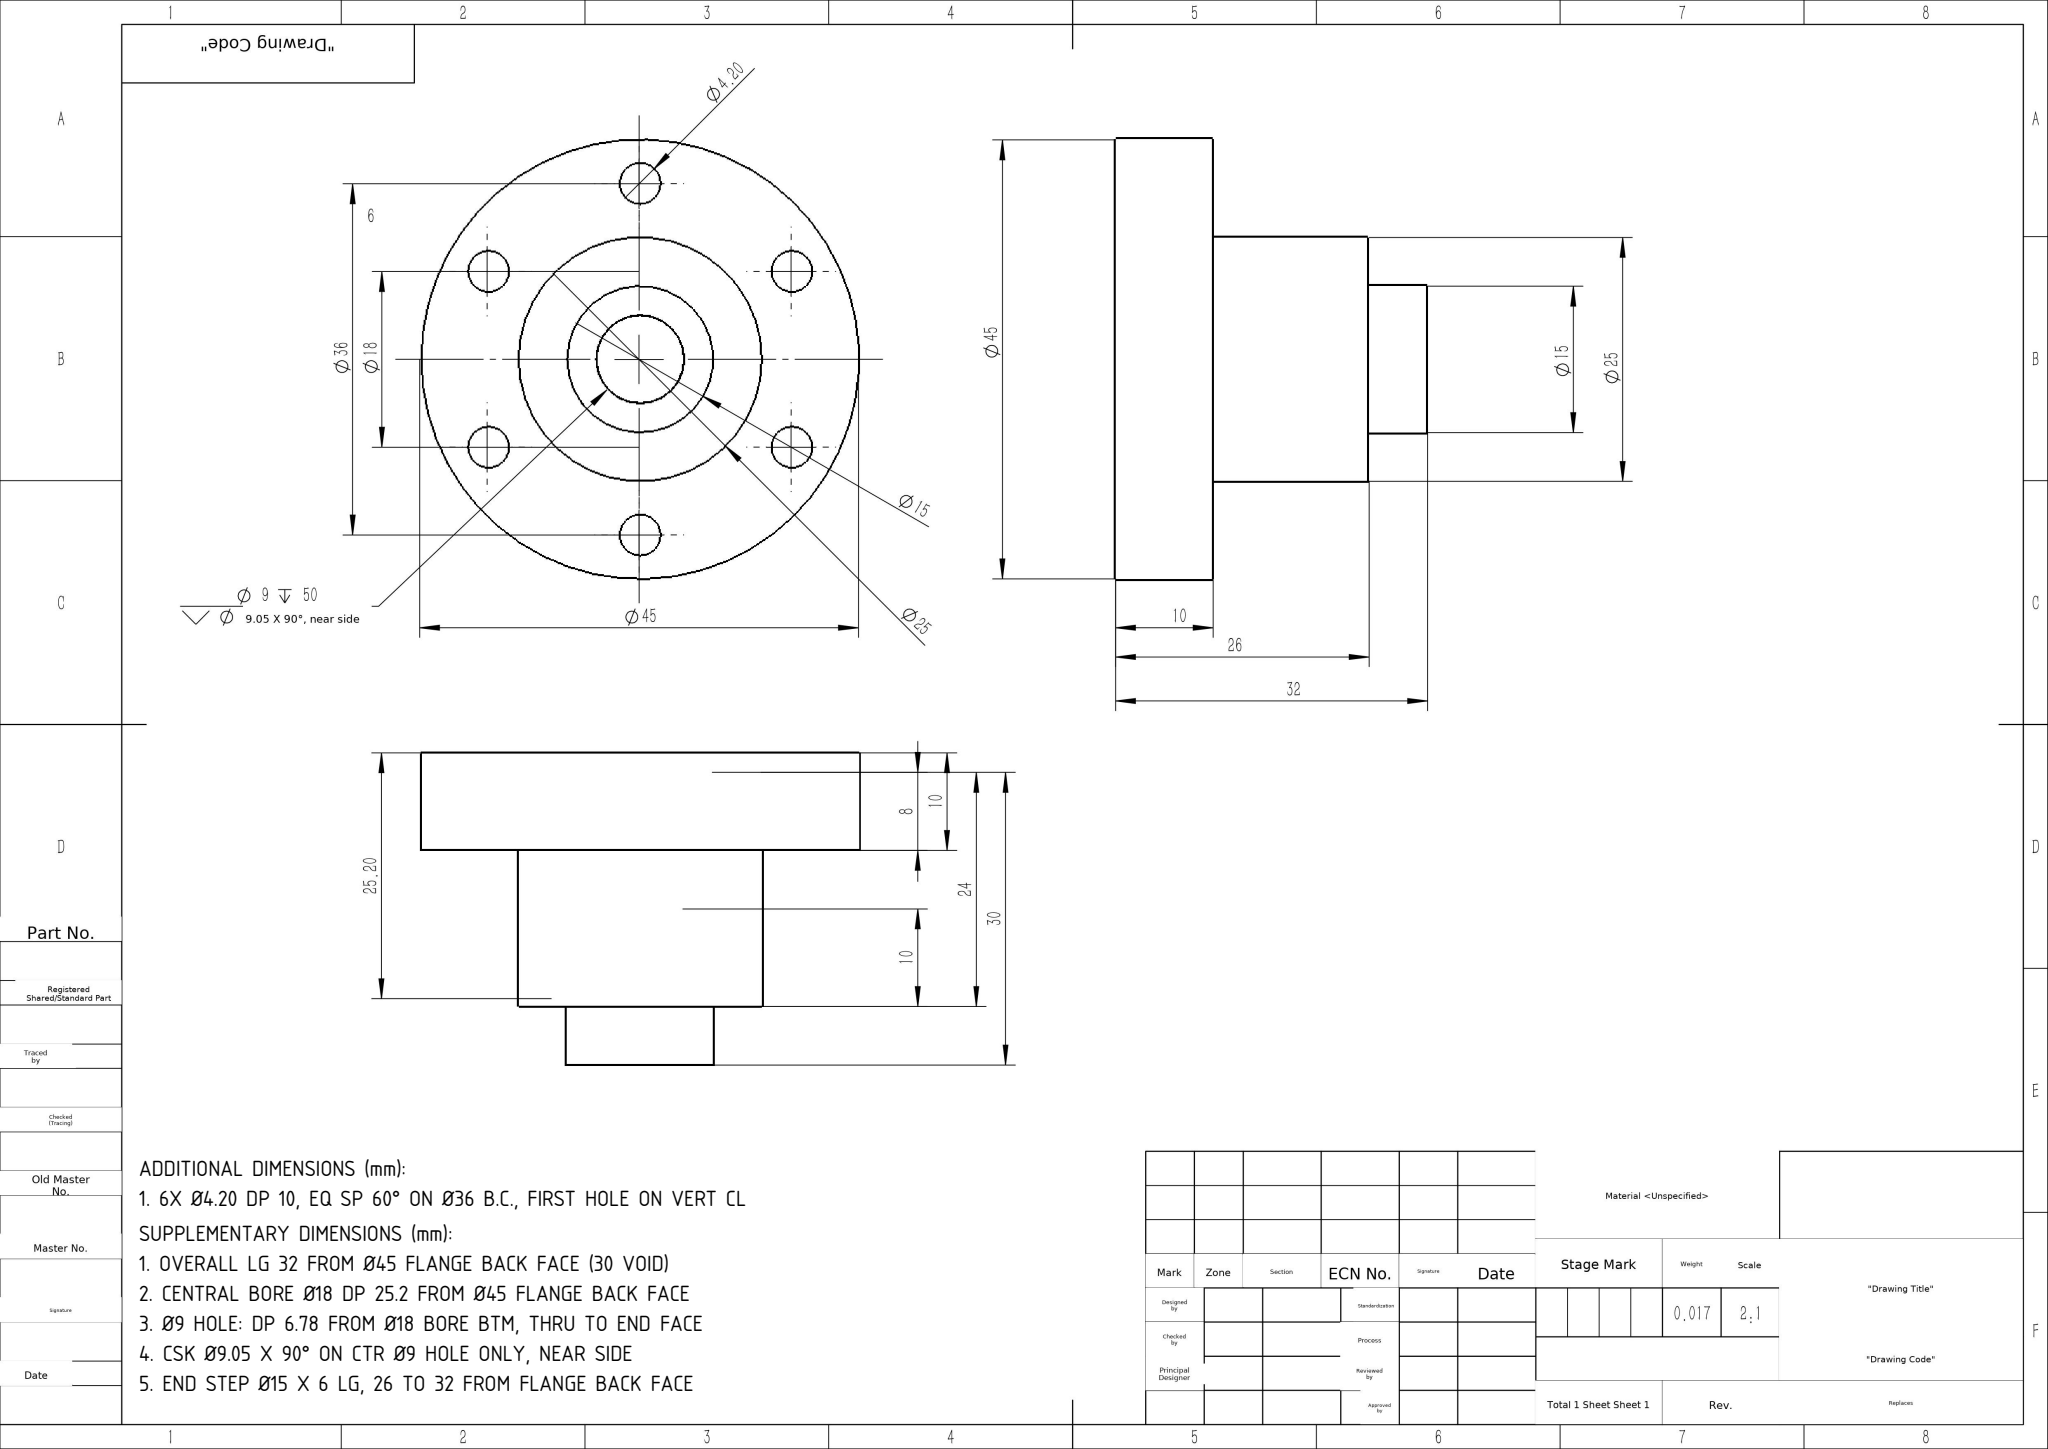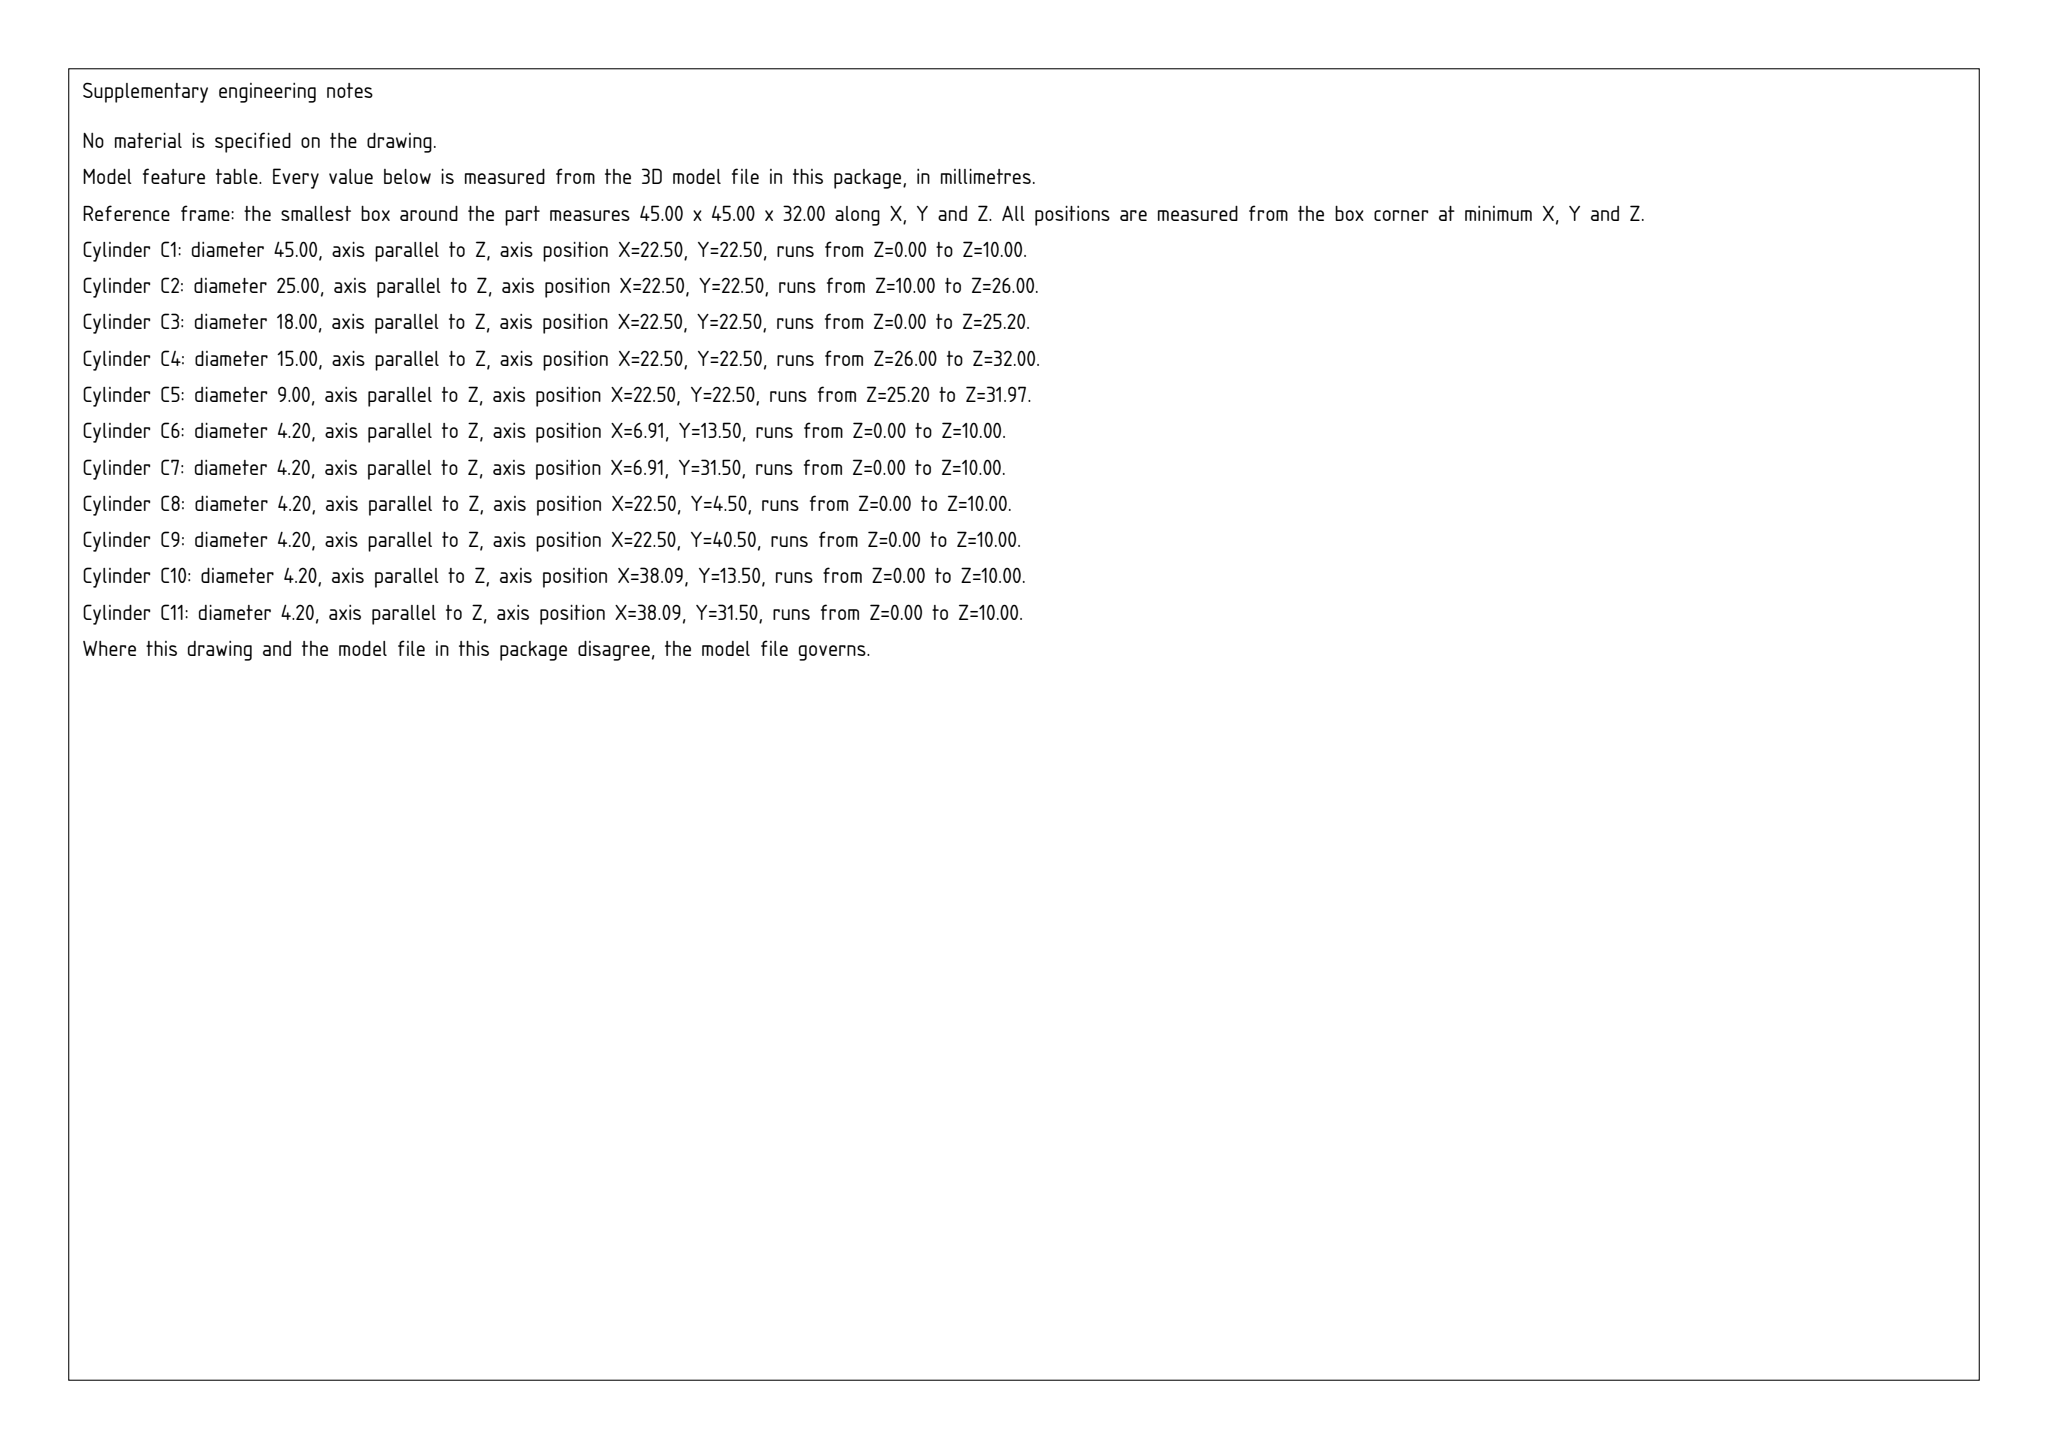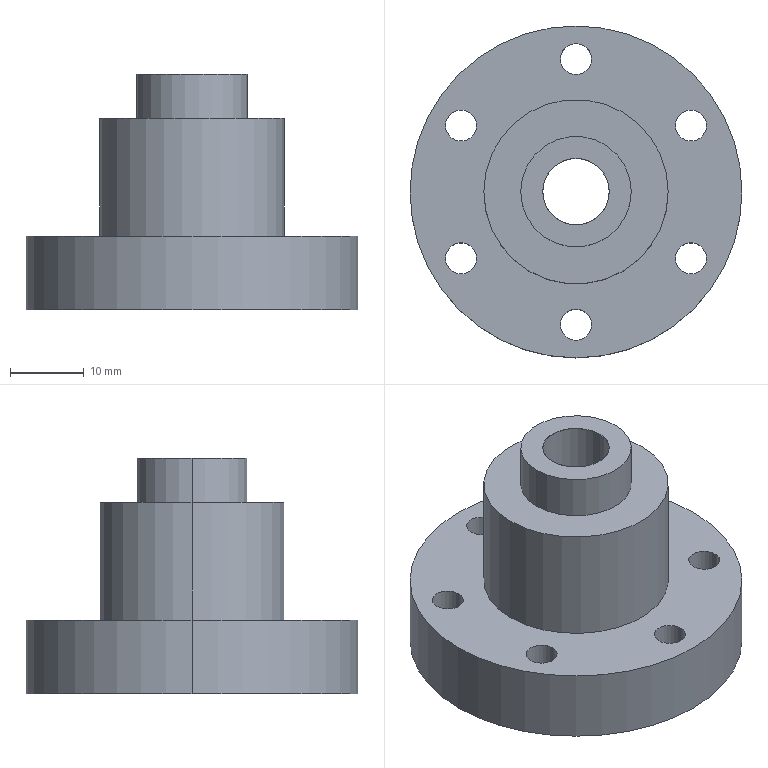Part | SolidWorks | mm | 1 solid | 29 faces | box 45 x 45 x 32 mm | volume 17142 mm3 | cylinder 22 | plane 5 | cone 2 | commonest cylinder face diameters 4.2 x12 18 x2 15 x2 9 x2 25 x2 45 x2
build123d program:
from build123d import *

# Parameters (mm, degrees)
SKETCH1_R                              = 22.5
BOSS_EXTRUDE1_DEPTH                    = 10
SKETCH2_R                              = 12.5
CUT_EXTRUDE1_DEPTH                     = 8
SKETCH3_R                              = 7.5
BOSS_EXTRUDE2_DEPTH                    = 30
SKETCH9_R                              = 2.1
CUT_EXTRUDE3_DEPTH                     = 46.128
M10X1_0_TAPPED_HOLE_DRILL1_D           = 9
M10X1_0_TAPPED_HOLE_DRILL1_DEPTH       = 50
M10X1_0_TAPPED_HOLE_DRILL1_CSINK_D     = 9.05
M10X1_0_TAPPED_HOLE_DRILL1_CSINK_ANGLE = 90
M10X1_0_TAPPED_HOLE_DRILL1_TIP         = 2.704
BOSS_EXTRUDE3_START                    = 24
SKETCH16_R                             = 12.5
BOSS_EXTRUDE3_DEPTH                    = 24
SKETCH15_R                             = 9
CUT_EXTRUDE5_DEPTH                     = 25.2
CUT_EXTRUDE6_START                     = -10
SKETCH17_R                             = 4.5
CUT_EXTRUDE6_DEPTH                     = 10


with BuildPart() as part:
    # Sketch1 → Boss-Extrude1 (new body)
    with BuildSketch(Plane.XY):
        Circle(SKETCH1_R)
    extrude(amount=BOSS_EXTRUDE1_DEPTH)

    # Sketch2 → Cut-Extrude1 (cut)
    with BuildSketch(Plane.XY.offset(10)):
        Circle(SKETCH2_R)
    extrude(amount=-CUT_EXTRUDE1_DEPTH, mode=Mode.SUBTRACT)

    # Sketch3 → Boss-Extrude2 (add)
    with BuildSketch(Plane.XY.offset(2)):
        Circle(SKETCH3_R)
    extrude(amount=BOSS_EXTRUDE2_DEPTH)

    # Sketch9 → Cut-Extrude3 (cut, through all)
    with BuildSketch(Plane(origin=(0, 0, 0), x_dir=(-1, 0, 0), z_dir=(0, 0, -1))):
        with Locations((0, 18)):
            Circle(SKETCH9_R)
        with Locations((15.588, 9)):
            Circle(SKETCH9_R)
        with Locations((15.588, -9)):
            Circle(SKETCH9_R)
        with Locations((0, -18)):
            Circle(SKETCH9_R)
        with Locations((-15.588, -9)):
            Circle(SKETCH9_R)
        with Locations((-15.588, 9)):
            Circle(SKETCH9_R)
    extrude(amount=-CUT_EXTRUDE3_DEPTH, mode=Mode.SUBTRACT)

    # M10X1.0 Tapped Hole Drill1
    with Locations(Plane.XY.offset(32)):
        with Locations((0, 0)):
            CounterSinkHole(M10X1_0_TAPPED_HOLE_DRILL1_D / 2, M10X1_0_TAPPED_HOLE_DRILL1_CSINK_D / 2, depth=M10X1_0_TAPPED_HOLE_DRILL1_DEPTH, counter_sink_angle=M10X1_0_TAPPED_HOLE_DRILL1_CSINK_ANGLE)
            with Locations((0, 0, -(M10X1_0_TAPPED_HOLE_DRILL1_DEPTH + M10X1_0_TAPPED_HOLE_DRILL1_TIP / 2))):  # 118° drill point
                Cone(0, M10X1_0_TAPPED_HOLE_DRILL1_D / 2, M10X1_0_TAPPED_HOLE_DRILL1_TIP, mode=Mode.SUBTRACT)

    # Sketch16 → Boss-Extrude3 (add)
    with BuildSketch(Plane.XY.offset(2).offset(BOSS_EXTRUDE3_START)):
        Circle(SKETCH16_R)
    extrude(amount=-BOSS_EXTRUDE3_DEPTH)

    # Sketch15 → Cut-Extrude5 (cut)
    with BuildSketch(Plane(origin=(0, 0, 0), x_dir=(-1, 0, 0), z_dir=(0, 0, -1))):
        Circle(SKETCH15_R)
    extrude(amount=-CUT_EXTRUDE5_DEPTH, mode=Mode.SUBTRACT)

    # Sketch17 → Cut-Extrude6 (cut)
    with BuildSketch(Plane.XY.offset(26).offset(CUT_EXTRUDE6_START)):
        Circle(SKETCH17_R)
    extrude(amount=CUT_EXTRUDE6_DEPTH, mode=Mode.SUBTRACT)


solid = part.part
STEP:
#1=CARTESIAN_POINT('',(9.,0.,25.2));
#2=VERTEX_POINT('',#1);
#3=CARTESIAN_POINT('',(-9.,0.,25.2));
#4=VERTEX_POINT('',#3);
#5=CARTESIAN_POINT('',(0.,0.,25.2));
#6=DIRECTION('',(0.,0.,-1.));
#7=DIRECTION('',(-1.,0.,0.));
#8=AXIS2_PLACEMENT_3D('',#5,#6,#7);
#9=CIRCLE('',#8,9.);
#10=EDGE_CURVE('',#2,#4,#9,.T.);
#11=ORIENTED_EDGE('',*,*,#10,.F.);
#12=CARTESIAN_POINT('',(9.,0.,0.));
#13=VERTEX_POINT('',#12);
#14=CARTESIAN_POINT('',(9.,0.,25.2));
#15=DIRECTION('',(0.,0.,-1.));
#16=VECTOR('',#15,1000.);
#17=LINE('',#14,#16);
#18=EDGE_CURVE('',#2,#13,#17,.T.);
#19=ORIENTED_EDGE('',*,*,#18,.T.);
#20=CARTESIAN_POINT('',(-9.,0.,0.));
#21=VERTEX_POINT('',#20);
#22=CARTESIAN_POINT('',(0.,0.,0.));
#23=DIRECTION('',(0.,0.,-1.));
#24=DIRECTION('',(-1.,0.,0.));
#25=AXIS2_PLACEMENT_3D('',#22,#23,#24);
#26=CIRCLE('',#25,9.);
#27=EDGE_CURVE('',#13,#21,#26,.T.);
#28=ORIENTED_EDGE('',*,*,#27,.T.);
#29=CARTESIAN_POINT('',(-9.,0.,25.2));
#30=DIRECTION('',(0.,0.,-1.));
#31=VECTOR('',#30,1000.);
#32=LINE('',#29,#31);
#33=EDGE_CURVE('',#4,#21,#32,.T.);
#34=ORIENTED_EDGE('',*,*,#33,.F.);
#35=EDGE_LOOP('',(#11,#19,#28,#34));
#36=FACE_OUTER_BOUND('',#35,.T.);
#37=CARTESIAN_POINT('',(0.,0.,25.2));
#38=DIRECTION('',(0.,0.,-1.));
#39=DIRECTION('',(-1.,0.,0.));
#40=AXIS2_PLACEMENT_3D('',#37,#38,#39);
#41=CYLINDRICAL_SURFACE('',#40,9.);
#42=ADVANCED_FACE('',(#36),#41,.F.);
#43=CARTESIAN_POINT('',(7.5,0.,32.));
#44=VERTEX_POINT('',#43);
#45=CARTESIAN_POINT('',(-7.5,0.,32.));
#46=VERTEX_POINT('',#45);
#47=CARTESIAN_POINT('',(0.,0.,32.));
#48=DIRECTION('',(0.,0.,1.));
#49=DIRECTION('',(1.,0.,0.));
#50=AXIS2_PLACEMENT_3D('',#47,#48,#49);
#51=CIRCLE('',#50,7.5);
#52=EDGE_CURVE('',#44,#46,#51,.T.);
#53=ORIENTED_EDGE('',*,*,#52,.F.);
#54=CARTESIAN_POINT('',(7.5,0.,26.));
#55=VERTEX_POINT('',#54);
#56=CARTESIAN_POINT('',(7.5,0.,32.));
#57=DIRECTION('',(0.,0.,-1.));
#58=VECTOR('',#57,1000.);
#59=LINE('',#56,#58);
#60=EDGE_CURVE('',#44,#55,#59,.T.);
#61=ORIENTED_EDGE('',*,*,#60,.T.);
#62=CARTESIAN_POINT('',(-7.5,0.,26.));
#63=VERTEX_POINT('',#62);
#64=CARTESIAN_POINT('',(0.,0.,26.));
#65=DIRECTION('',(0.,0.,1.));
#66=DIRECTION('',(1.,0.,0.));
#67=AXIS2_PLACEMENT_3D('',#64,#65,#66);
#68=CIRCLE('',#67,7.5);
#69=EDGE_CURVE('',#55,#63,#68,.T.);
#70=ORIENTED_EDGE('',*,*,#69,.T.);
#71=CARTESIAN_POINT('',(-7.5,0.,32.));
#72=DIRECTION('',(0.,0.,-1.));
#73=VECTOR('',#72,1000.);
#74=LINE('',#71,#73);
#75=EDGE_CURVE('',#46,#63,#74,.T.);
#76=ORIENTED_EDGE('',*,*,#75,.F.);
#77=EDGE_LOOP('',(#53,#61,#70,#76));
#78=FACE_OUTER_BOUND('',#77,.T.);
#79=CARTESIAN_POINT('',(0.,0.,32.));
#80=DIRECTION('',(0.,0.,-1.));
#81=DIRECTION('',(-1.,0.,0.));
#82=AXIS2_PLACEMENT_3D('',#79,#80,#81);
#83=CYLINDRICAL_SURFACE('',#82,7.5);
#84=ADVANCED_FACE('',(#78),#83,.T.);
#85=CARTESIAN_POINT('',(4.5,0.,25.2));
#86=VERTEX_POINT('',#85);
#87=CARTESIAN_POINT('',(-4.5,0.,25.2));
#88=VERTEX_POINT('',#87);
#89=CARTESIAN_POINT('',(0.,0.,25.2));
#90=DIRECTION('',(0.,0.,-1.));
#91=DIRECTION('',(-1.,0.,0.));
#92=AXIS2_PLACEMENT_3D('',#89,#90,#91);
#93=CIRCLE('',#92,4.5);
#94=EDGE_CURVE('',#86,#88,#93,.T.);
#95=ORIENTED_EDGE('',*,*,#94,.T.);
#96=CARTESIAN_POINT('',(-4.5,0.,31.975));
#97=VERTEX_POINT('',#96);
#98=CARTESIAN_POINT('',(-4.5,0.,32.));
#99=DIRECTION('',(0.,0.,1.));
#100=VECTOR('',#99,1000.);
#101=LINE('',#98,#100);
#102=EDGE_CURVE('',#88,#97,#101,.T.);
#103=ORIENTED_EDGE('',*,*,#102,.T.);
#104=CARTESIAN_POINT('',(4.5,0.,31.975));
#105=VERTEX_POINT('',#104);
#106=CARTESIAN_POINT('',(0.,0.,31.975));
#107=DIRECTION('',(0.,0.,1.));
#108=DIRECTION('',(1.,0.,0.));
#109=AXIS2_PLACEMENT_3D('',#106,#107,#108);
#110=CIRCLE('',#109,4.5);
#111=EDGE_CURVE('',#97,#105,#110,.T.);
#112=ORIENTED_EDGE('',*,*,#111,.T.);
#113=CARTESIAN_POINT('',(4.5,0.,32.));
#114=DIRECTION('',(0.,0.,1.));
#115=VECTOR('',#114,1000.);
#116=LINE('',#113,#115);
#117=EDGE_CURVE('',#86,#105,#116,.T.);
#118=ORIENTED_EDGE('',*,*,#117,.F.);
#119=EDGE_LOOP('',(#95,#103,#112,#118));
#120=FACE_OUTER_BOUND('',#119,.T.);
#121=CARTESIAN_POINT('',(0.,0.,32.));
#122=DIRECTION('',(0.,0.,1.));
#123=DIRECTION('',(1.,0.,0.));
#124=AXIS2_PLACEMENT_3D('',#121,#122,#123);
#125=CYLINDRICAL_SURFACE('',#124,4.5);
#126=ADVANCED_FACE('',(#120),#125,.F.);
#127=ORIENTED_EDGE('',*,*,#111,.F.);
#128=CARTESIAN_POINT('',(-4.525,0.,32.));
#129=VERTEX_POINT('',#128);
#130=CARTESIAN_POINT('',(-4.525,0.,32.));
#131=DIRECTION('',(-0.7071,0.,0.7071));
#132=VECTOR('',#131,1000.);
#133=LINE('',#130,#132);
#134=EDGE_CURVE('',#97,#129,#133,.T.);
#135=ORIENTED_EDGE('',*,*,#134,.T.);
#136=CARTESIAN_POINT('',(4.525,0.,32.));
#137=VERTEX_POINT('',#136);
#138=CARTESIAN_POINT('',(0.,0.,32.));
#139=DIRECTION('',(0.,0.,1.));
#140=DIRECTION('',(1.,0.,0.));
#141=AXIS2_PLACEMENT_3D('',#138,#139,#140);
#142=CIRCLE('',#141,4.525);
#143=EDGE_CURVE('',#129,#137,#142,.T.);
#144=ORIENTED_EDGE('',*,*,#143,.T.);
#145=CARTESIAN_POINT('',(4.525,0.,32.));
#146=DIRECTION('',(0.7071,0.,0.7071));
#147=VECTOR('',#146,1000.);
#148=LINE('',#145,#147);
#149=EDGE_CURVE('',#105,#137,#148,.T.);
#150=ORIENTED_EDGE('',*,*,#149,.F.);
#151=EDGE_LOOP('',(#127,#135,#144,#150));
#152=FACE_OUTER_BOUND('',#151,.T.);
#153=CARTESIAN_POINT('',(0.,0.,32.));
#154=DIRECTION('',(0.,0.,1.));
#155=DIRECTION('',(1.,0.,0.));
#156=AXIS2_PLACEMENT_3D('',#153,#154,#155);
#157=CONICAL_SURFACE('',#156,4.525,0.7854);
#158=ADVANCED_FACE('',(#152),#157,.F.);
#159=CARTESIAN_POINT('',(12.5,0.,26.));
#160=VERTEX_POINT('',#159);
#161=CARTESIAN_POINT('',(-12.5,0.,26.));
#162=VERTEX_POINT('',#161);
#163=CARTESIAN_POINT('',(0.,0.,26.));
#164=DIRECTION('',(0.,0.,1.));
#165=DIRECTION('',(1.,0.,0.));
#166=AXIS2_PLACEMENT_3D('',#163,#164,#165);
#167=CIRCLE('',#166,12.5);
#168=EDGE_CURVE('',#160,#162,#167,.T.);
#169=ORIENTED_EDGE('',*,*,#168,.F.);
#170=CARTESIAN_POINT('',(12.5,0.,10.));
#171=VERTEX_POINT('',#170);
#172=CARTESIAN_POINT('',(12.5,0.,26.));
#173=DIRECTION('',(0.,0.,-1.));
#174=VECTOR('',#173,1000.);
#175=LINE('',#172,#174);
#176=EDGE_CURVE('',#160,#171,#175,.T.);
#177=ORIENTED_EDGE('',*,*,#176,.T.);
#178=CARTESIAN_POINT('',(-12.5,0.,10.));
#179=VERTEX_POINT('',#178);
#180=CARTESIAN_POINT('',(0.,0.,10.));
#181=DIRECTION('',(0.,0.,1.));
#182=DIRECTION('',(1.,0.,0.));
#183=AXIS2_PLACEMENT_3D('',#180,#181,#182);
#184=CIRCLE('',#183,12.5);
#185=EDGE_CURVE('',#171,#179,#184,.T.);
#186=ORIENTED_EDGE('',*,*,#185,.T.);
#187=CARTESIAN_POINT('',(-12.5,0.,26.));
#188=DIRECTION('',(0.,0.,-1.));
#189=VECTOR('',#188,1000.);
#190=LINE('',#187,#189);
#191=EDGE_CURVE('',#162,#179,#190,.T.);
#192=ORIENTED_EDGE('',*,*,#191,.F.);
#193=EDGE_LOOP('',(#169,#177,#186,#192));
#194=FACE_OUTER_BOUND('',#193,.T.);
#195=CARTESIAN_POINT('',(0.,0.,26.));
#196=DIRECTION('',(0.,0.,-1.));
#197=DIRECTION('',(-1.,0.,0.));
#198=AXIS2_PLACEMENT_3D('',#195,#196,#197);
#199=CYLINDRICAL_SURFACE('',#198,12.5);
#200=ADVANCED_FACE('',(#194),#199,.T.);
#201=CARTESIAN_POINT('',(-2.1,18.,10.));
#202=VERTEX_POINT('',#201);
#203=CARTESIAN_POINT('',(2.1,18.,10.));
#204=VERTEX_POINT('',#203);
#205=CARTESIAN_POINT('',(0.,18.,10.));
#206=DIRECTION('',(0.,0.,1.));
#207=DIRECTION('',(1.,0.,0.));
#208=AXIS2_PLACEMENT_3D('',#205,#206,#207);
#209=CIRCLE('',#208,2.1);
#210=EDGE_CURVE('',#202,#204,#209,.T.);
#211=ORIENTED_EDGE('',*,*,#210,.T.);
#212=CARTESIAN_POINT('',(2.1,18.,0.));
#213=VERTEX_POINT('',#212);
#214=CARTESIAN_POINT('',(2.1,18.,32.));
#215=DIRECTION('',(0.,0.,-1.));
#216=VECTOR('',#215,1000.);
#217=LINE('',#214,#216);
#218=EDGE_CURVE('',#204,#213,#217,.T.);
#219=ORIENTED_EDGE('',*,*,#218,.T.);
#220=CARTESIAN_POINT('',(-2.1,18.,0.));
#221=VERTEX_POINT('',#220);
#222=CARTESIAN_POINT('',(0.,18.,0.));
#223=DIRECTION('',(0.,0.,-1.));
#224=DIRECTION('',(-1.,0.,0.));
#225=AXIS2_PLACEMENT_3D('',#222,#223,#224);
#226=CIRCLE('',#225,2.1);
#227=EDGE_CURVE('',#213,#221,#226,.T.);
#228=ORIENTED_EDGE('',*,*,#227,.T.);
#229=CARTESIAN_POINT('',(-2.1,18.,32.));
#230=DIRECTION('',(0.,0.,-1.));
#231=VECTOR('',#230,1000.);
#232=LINE('',#229,#231);
#233=EDGE_CURVE('',#202,#221,#232,.T.);
#234=ORIENTED_EDGE('',*,*,#233,.F.);
#235=EDGE_LOOP('',(#211,#219,#228,#234));
#236=FACE_OUTER_BOUND('',#235,.T.);
#237=CARTESIAN_POINT('',(0.,18.,32.));
#238=DIRECTION('',(0.,0.,-1.));
#239=DIRECTION('',(-1.,0.,0.));
#240=AXIS2_PLACEMENT_3D('',#237,#238,#239);
#241=CYLINDRICAL_SURFACE('',#240,2.1);
#242=ADVANCED_FACE('',(#236),#241,.F.);
#243=CARTESIAN_POINT('',(13.488,9.,10.));
#244=VERTEX_POINT('',#243);
#245=CARTESIAN_POINT('',(17.688,9.,10.));
#246=VERTEX_POINT('',#245);
#247=CARTESIAN_POINT('',(15.588,9.,10.));
#248=DIRECTION('',(0.,0.,1.));
#249=DIRECTION('',(1.,0.,0.));
#250=AXIS2_PLACEMENT_3D('',#247,#248,#249);
#251=CIRCLE('',#250,2.1);
#252=EDGE_CURVE('',#244,#246,#251,.T.);
#253=ORIENTED_EDGE('',*,*,#252,.T.);
#254=CARTESIAN_POINT('',(17.688,9.,0.));
#255=VERTEX_POINT('',#254);
#256=CARTESIAN_POINT('',(17.688,9.,32.));
#257=DIRECTION('',(0.,0.,-1.));
#258=VECTOR('',#257,1000.);
#259=LINE('',#256,#258);
#260=EDGE_CURVE('',#246,#255,#259,.T.);
#261=ORIENTED_EDGE('',*,*,#260,.T.);
#262=CARTESIAN_POINT('',(13.488,9.,0.));
#263=VERTEX_POINT('',#262);
#264=CARTESIAN_POINT('',(15.588,9.,0.));
#265=DIRECTION('',(0.,0.,-1.));
#266=DIRECTION('',(-1.,0.,0.));
#267=AXIS2_PLACEMENT_3D('',#264,#265,#266);
#268=CIRCLE('',#267,2.1);
#269=EDGE_CURVE('',#255,#263,#268,.T.);
#270=ORIENTED_EDGE('',*,*,#269,.T.);
#271=CARTESIAN_POINT('',(13.488,9.,32.));
#272=DIRECTION('',(0.,0.,-1.));
#273=VECTOR('',#272,1000.);
#274=LINE('',#271,#273);
#275=EDGE_CURVE('',#244,#263,#274,.T.);
#276=ORIENTED_EDGE('',*,*,#275,.F.);
#277=EDGE_LOOP('',(#253,#261,#270,#276));
#278=FACE_OUTER_BOUND('',#277,.T.);
#279=CARTESIAN_POINT('',(15.588,9.,32.));
#280=DIRECTION('',(0.,0.,-1.));
#281=DIRECTION('',(-1.,0.,0.));
#282=AXIS2_PLACEMENT_3D('',#279,#280,#281);
#283=CYLINDRICAL_SURFACE('',#282,2.1);
#284=ADVANCED_FACE('',(#278),#283,.F.);
#285=CARTESIAN_POINT('',(13.488,-9.,10.));
#286=VERTEX_POINT('',#285);
#287=CARTESIAN_POINT('',(17.688,-9.,10.));
#288=VERTEX_POINT('',#287);
#289=CARTESIAN_POINT('',(15.588,-9.,10.));
#290=DIRECTION('',(0.,0.,1.));
#291=DIRECTION('',(1.,0.,0.));
#292=AXIS2_PLACEMENT_3D('',#289,#290,#291);
#293=CIRCLE('',#292,2.1);
#294=EDGE_CURVE('',#286,#288,#293,.T.);
#295=ORIENTED_EDGE('',*,*,#294,.T.);
#296=CARTESIAN_POINT('',(17.688,-9.,0.));
#297=VERTEX_POINT('',#296);
#298=CARTESIAN_POINT('',(17.688,-9.,32.));
#299=DIRECTION('',(0.,0.,-1.));
#300=VECTOR('',#299,1000.);
#301=LINE('',#298,#300);
#302=EDGE_CURVE('',#288,#297,#301,.T.);
#303=ORIENTED_EDGE('',*,*,#302,.T.);
#304=CARTESIAN_POINT('',(13.488,-9.,0.));
#305=VERTEX_POINT('',#304);
#306=CARTESIAN_POINT('',(15.588,-9.,0.));
#307=DIRECTION('',(0.,0.,-1.));
#308=DIRECTION('',(-1.,0.,0.));
#309=AXIS2_PLACEMENT_3D('',#306,#307,#308);
#310=CIRCLE('',#309,2.1);
#311=EDGE_CURVE('',#297,#305,#310,.T.);
#312=ORIENTED_EDGE('',*,*,#311,.T.);
#313=CARTESIAN_POINT('',(13.488,-9.,32.));
#314=DIRECTION('',(0.,0.,-1.));
#315=VECTOR('',#314,1000.);
#316=LINE('',#313,#315);
#317=EDGE_CURVE('',#286,#305,#316,.T.);
#318=ORIENTED_EDGE('',*,*,#317,.F.);
#319=EDGE_LOOP('',(#295,#303,#312,#318));
#320=FACE_OUTER_BOUND('',#319,.T.);
#321=CARTESIAN_POINT('',(15.588,-9.,32.));
#322=DIRECTION('',(0.,0.,-1.));
#323=DIRECTION('',(-1.,0.,0.));
#324=AXIS2_PLACEMENT_3D('',#321,#322,#323);
#325=CYLINDRICAL_SURFACE('',#324,2.1);
#326=ADVANCED_FACE('',(#320),#325,.F.);
#327=CARTESIAN_POINT('',(-2.1,-18.,10.));
#328=VERTEX_POINT('',#327);
#329=CARTESIAN_POINT('',(2.1,-18.,10.));
#330=VERTEX_POINT('',#329);
#331=CARTESIAN_POINT('',(0.,-18.,10.));
#332=DIRECTION('',(0.,0.,1.));
#333=DIRECTION('',(1.,0.,0.));
#334=AXIS2_PLACEMENT_3D('',#331,#332,#333);
#335=CIRCLE('',#334,2.1);
#336=EDGE_CURVE('',#328,#330,#335,.T.);
#337=ORIENTED_EDGE('',*,*,#336,.T.);
#338=CARTESIAN_POINT('',(2.1,-18.,0.));
#339=VERTEX_POINT('',#338);
#340=CARTESIAN_POINT('',(2.1,-18.,32.));
#341=DIRECTION('',(0.,0.,-1.));
#342=VECTOR('',#341,1000.);
#343=LINE('',#340,#342);
#344=EDGE_CURVE('',#330,#339,#343,.T.);
#345=ORIENTED_EDGE('',*,*,#344,.T.);
#346=CARTESIAN_POINT('',(-2.1,-18.,0.));
#347=VERTEX_POINT('',#346);
#348=CARTESIAN_POINT('',(0.,-18.,0.));
#349=DIRECTION('',(0.,0.,-1.));
#350=DIRECTION('',(-1.,0.,0.));
#351=AXIS2_PLACEMENT_3D('',#348,#349,#350);
#352=CIRCLE('',#351,2.1);
#353=EDGE_CURVE('',#339,#347,#352,.T.);
#354=ORIENTED_EDGE('',*,*,#353,.T.);
#355=CARTESIAN_POINT('',(-2.1,-18.,32.));
#356=DIRECTION('',(0.,0.,-1.));
#357=VECTOR('',#356,1000.);
#358=LINE('',#355,#357);
#359=EDGE_CURVE('',#328,#347,#358,.T.);
#360=ORIENTED_EDGE('',*,*,#359,.F.);
#361=EDGE_LOOP('',(#337,#345,#354,#360));
#362=FACE_OUTER_BOUND('',#361,.T.);
#363=CARTESIAN_POINT('',(0.,-18.,32.));
#364=DIRECTION('',(0.,0.,-1.));
#365=DIRECTION('',(-1.,0.,0.));
#366=AXIS2_PLACEMENT_3D('',#363,#364,#365);
#367=CYLINDRICAL_SURFACE('',#366,2.1);
#368=ADVANCED_FACE('',(#362),#367,.F.);
#369=CARTESIAN_POINT('',(-17.688,-9.,10.));
#370=VERTEX_POINT('',#369);
#371=CARTESIAN_POINT('',(-13.488,-9.,10.));
#372=VERTEX_POINT('',#371);
#373=CARTESIAN_POINT('',(-15.588,-9.,10.));
#374=DIRECTION('',(0.,0.,1.));
#375=DIRECTION('',(1.,0.,0.));
#376=AXIS2_PLACEMENT_3D('',#373,#374,#375);
#377=CIRCLE('',#376,2.1);
#378=EDGE_CURVE('',#370,#372,#377,.T.);
#379=ORIENTED_EDGE('',*,*,#378,.T.);
#380=CARTESIAN_POINT('',(-13.488,-9.,0.));
#381=VERTEX_POINT('',#380);
#382=CARTESIAN_POINT('',(-13.488,-9.,32.));
#383=DIRECTION('',(0.,0.,-1.));
#384=VECTOR('',#383,1000.);
#385=LINE('',#382,#384);
#386=EDGE_CURVE('',#372,#381,#385,.T.);
#387=ORIENTED_EDGE('',*,*,#386,.T.);
#388=CARTESIAN_POINT('',(-17.688,-9.,0.));
#389=VERTEX_POINT('',#388);
#390=CARTESIAN_POINT('',(-15.588,-9.,0.));
#391=DIRECTION('',(0.,0.,-1.));
#392=DIRECTION('',(-1.,0.,0.));
#393=AXIS2_PLACEMENT_3D('',#390,#391,#392);
#394=CIRCLE('',#393,2.1);
#395=EDGE_CURVE('',#381,#389,#394,.T.);
#396=ORIENTED_EDGE('',*,*,#395,.T.);
#397=CARTESIAN_POINT('',(-17.688,-9.,32.));
#398=DIRECTION('',(0.,0.,-1.));
#399=VECTOR('',#398,1000.);
#400=LINE('',#397,#399);
#401=EDGE_CURVE('',#370,#389,#400,.T.);
#402=ORIENTED_EDGE('',*,*,#401,.F.);
#403=EDGE_LOOP('',(#379,#387,#396,#402));
#404=FACE_OUTER_BOUND('',#403,.T.);
#405=CARTESIAN_POINT('',(-15.588,-9.,32.));
#406=DIRECTION('',(0.,0.,-1.));
#407=DIRECTION('',(-1.,0.,0.));
#408=AXIS2_PLACEMENT_3D('',#405,#406,#407);
#409=CYLINDRICAL_SURFACE('',#408,2.1);
#410=ADVANCED_FACE('',(#404),#409,.F.);
#411=CARTESIAN_POINT('',(-17.688,9.,10.));
#412=VERTEX_POINT('',#411);
#413=CARTESIAN_POINT('',(-13.488,9.,10.));
#414=VERTEX_POINT('',#413);
#415=CARTESIAN_POINT('',(-15.588,9.,10.));
#416=DIRECTION('',(0.,0.,1.));
#417=DIRECTION('',(1.,0.,0.));
#418=AXIS2_PLACEMENT_3D('',#415,#416,#417);
#419=CIRCLE('',#418,2.1);
#420=EDGE_CURVE('',#412,#414,#419,.T.);
#421=ORIENTED_EDGE('',*,*,#420,.T.);
#422=CARTESIAN_POINT('',(-13.488,9.,0.));
#423=VERTEX_POINT('',#422);
#424=CARTESIAN_POINT('',(-13.488,9.,32.));
#425=DIRECTION('',(0.,0.,-1.));
#426=VECTOR('',#425,1000.);
#427=LINE('',#424,#426);
#428=EDGE_CURVE('',#414,#423,#427,.T.);
#429=ORIENTED_EDGE('',*,*,#428,.T.);
#430=CARTESIAN_POINT('',(-17.688,9.,0.));
#431=VERTEX_POINT('',#430);
#432=CARTESIAN_POINT('',(-15.588,9.,0.));
#433=DIRECTION('',(0.,0.,-1.));
#434=DIRECTION('',(-1.,0.,0.));
#435=AXIS2_PLACEMENT_3D('',#432,#433,#434);
#436=CIRCLE('',#435,2.1);
#437=EDGE_CURVE('',#423,#431,#436,.T.);
#438=ORIENTED_EDGE('',*,*,#437,.T.);
#439=CARTESIAN_POINT('',(-17.688,9.,32.));
#440=DIRECTION('',(0.,0.,-1.));
#441=VECTOR('',#440,1000.);
#442=LINE('',#439,#441);
#443=EDGE_CURVE('',#412,#431,#442,.T.);
#444=ORIENTED_EDGE('',*,*,#443,.F.);
#445=EDGE_LOOP('',(#421,#429,#438,#444));
#446=FACE_OUTER_BOUND('',#445,.T.);
#447=CARTESIAN_POINT('',(-15.588,9.,32.));
#448=DIRECTION('',(0.,0.,-1.));
#449=DIRECTION('',(-1.,0.,0.));
#450=AXIS2_PLACEMENT_3D('',#447,#448,#449);
#451=CYLINDRICAL_SURFACE('',#450,2.1);
#452=ADVANCED_FACE('',(#446),#451,.F.);
#453=CARTESIAN_POINT('',(22.5,0.,10.));
#454=VERTEX_POINT('',#453);
#455=CARTESIAN_POINT('',(-22.5,0.,10.));
#456=VERTEX_POINT('',#455);
#457=CARTESIAN_POINT('',(0.,0.,10.));
#458=DIRECTION('',(0.,0.,1.));
#459=DIRECTION('',(1.,0.,0.));
#460=AXIS2_PLACEMENT_3D('',#457,#458,#459);
#461=CIRCLE('',#460,22.5);
#462=EDGE_CURVE('',#454,#456,#461,.T.);
#463=ORIENTED_EDGE('',*,*,#462,.F.);
#464=CARTESIAN_POINT('',(22.5,0.,0.));
#465=VERTEX_POINT('',#464);
#466=CARTESIAN_POINT('',(22.5,0.,10.));
#467=DIRECTION('',(0.,0.,-1.));
#468=VECTOR('',#467,1000.);
#469=LINE('',#466,#468);
#470=EDGE_CURVE('',#454,#465,#469,.T.);
#471=ORIENTED_EDGE('',*,*,#470,.T.);
#472=CARTESIAN_POINT('',(-22.5,0.,0.));
#473=VERTEX_POINT('',#472);
#474=CARTESIAN_POINT('',(0.,0.,0.));
#475=DIRECTION('',(0.,0.,1.));
#476=DIRECTION('',(1.,0.,0.));
#477=AXIS2_PLACEMENT_3D('',#474,#475,#476);
#478=CIRCLE('',#477,22.5);
#479=EDGE_CURVE('',#465,#473,#478,.T.);
#480=ORIENTED_EDGE('',*,*,#479,.T.);
#481=CARTESIAN_POINT('',(-22.5,0.,10.));
#482=DIRECTION('',(0.,0.,-1.));
#483=VECTOR('',#482,1000.);
#484=LINE('',#481,#483);
#485=EDGE_CURVE('',#456,#473,#484,.T.);
#486=ORIENTED_EDGE('',*,*,#485,.F.);
#487=EDGE_LOOP('',(#463,#471,#480,#486));
#488=FACE_OUTER_BOUND('',#487,.T.);
#489=CARTESIAN_POINT('',(0.,0.,10.));
#490=DIRECTION('',(0.,0.,-1.));
#491=DIRECTION('',(-1.,0.,0.));
#492=AXIS2_PLACEMENT_3D('',#489,#490,#491);
#493=CYLINDRICAL_SURFACE('',#492,22.5);
#494=ADVANCED_FACE('',(#488),#493,.T.);
#495=ORIENTED_EDGE('',*,*,#470,.F.);
#496=CARTESIAN_POINT('',(0.,0.,10.));
#497=DIRECTION('',(0.,0.,1.));
#498=DIRECTION('',(1.,0.,0.));
#499=AXIS2_PLACEMENT_3D('',#496,#497,#498);
#500=CIRCLE('',#499,22.5);
#501=EDGE_CURVE('',#456,#454,#500,.T.);
#502=ORIENTED_EDGE('',*,*,#501,.F.);
#503=ORIENTED_EDGE('',*,*,#485,.T.);
#504=CARTESIAN_POINT('',(0.,0.,0.));
#505=DIRECTION('',(0.,0.,1.));
#506=DIRECTION('',(1.,0.,0.));
#507=AXIS2_PLACEMENT_3D('',#504,#505,#506);
#508=CIRCLE('',#507,22.5);
#509=EDGE_CURVE('',#473,#465,#508,.T.);
#510=ORIENTED_EDGE('',*,*,#509,.T.);
#511=EDGE_LOOP('',(#495,#502,#503,#510));
#512=FACE_OUTER_BOUND('',#511,.T.);
#513=CARTESIAN_POINT('',(0.,0.,10.));
#514=DIRECTION('',(0.,0.,-1.));
#515=DIRECTION('',(-1.,0.,0.));
#516=AXIS2_PLACEMENT_3D('',#513,#514,#515);
#517=CYLINDRICAL_SURFACE('',#516,22.5);
#518=ADVANCED_FACE('',(#512),#517,.T.);
#519=ORIENTED_EDGE('',*,*,#210,.F.);
#520=CARTESIAN_POINT('',(0.,18.,10.));
#521=DIRECTION('',(0.,0.,1.));
#522=DIRECTION('',(1.,0.,0.));
#523=AXIS2_PLACEMENT_3D('',#520,#521,#522);
#524=CIRCLE('',#523,2.1);
#525=EDGE_CURVE('',#204,#202,#524,.T.);
#526=ORIENTED_EDGE('',*,*,#525,.F.);
#527=EDGE_LOOP('',(#519,#526));
#528=FACE_BOUND('',#527,.T.);
#529=ORIENTED_EDGE('',*,*,#252,.F.);
#530=CARTESIAN_POINT('',(15.588,9.,10.));
#531=DIRECTION('',(0.,0.,1.));
#532=DIRECTION('',(1.,0.,0.));
#533=AXIS2_PLACEMENT_3D('',#530,#531,#532);
#534=CIRCLE('',#533,2.1);
#535=EDGE_CURVE('',#246,#244,#534,.T.);
#536=ORIENTED_EDGE('',*,*,#535,.F.);
#537=EDGE_LOOP('',(#529,#536));
#538=FACE_BOUND('',#537,.T.);
#539=ORIENTED_EDGE('',*,*,#294,.F.);
#540=CARTESIAN_POINT('',(15.588,-9.,10.));
#541=DIRECTION('',(0.,0.,1.));
#542=DIRECTION('',(1.,0.,0.));
#543=AXIS2_PLACEMENT_3D('',#540,#541,#542);
#544=CIRCLE('',#543,2.1);
#545=EDGE_CURVE('',#288,#286,#544,.T.);
#546=ORIENTED_EDGE('',*,*,#545,.F.);
#547=EDGE_LOOP('',(#539,#546));
#548=FACE_BOUND('',#547,.T.);
#549=ORIENTED_EDGE('',*,*,#336,.F.);
#550=CARTESIAN_POINT('',(0.,-18.,10.));
#551=DIRECTION('',(0.,0.,1.));
#552=DIRECTION('',(1.,0.,0.));
#553=AXIS2_PLACEMENT_3D('',#550,#551,#552);
#554=CIRCLE('',#553,2.1);
#555=EDGE_CURVE('',#330,#328,#554,.T.);
#556=ORIENTED_EDGE('',*,*,#555,.F.);
#557=EDGE_LOOP('',(#549,#556));
#558=FACE_BOUND('',#557,.T.);
#559=ORIENTED_EDGE('',*,*,#378,.F.);
#560=CARTESIAN_POINT('',(-15.588,-9.,10.));
#561=DIRECTION('',(0.,0.,1.));
#562=DIRECTION('',(1.,0.,0.));
#563=AXIS2_PLACEMENT_3D('',#560,#561,#562);
#564=CIRCLE('',#563,2.1);
#565=EDGE_CURVE('',#372,#370,#564,.T.);
#566=ORIENTED_EDGE('',*,*,#565,.F.);
#567=EDGE_LOOP('',(#559,#566));
#568=FACE_BOUND('',#567,.T.);
#569=ORIENTED_EDGE('',*,*,#420,.F.);
#570=CARTESIAN_POINT('',(-15.588,9.,10.));
#571=DIRECTION('',(0.,0.,1.));
#572=DIRECTION('',(1.,0.,0.));
#573=AXIS2_PLACEMENT_3D('',#570,#571,#572);
#574=CIRCLE('',#573,2.1);
#575=EDGE_CURVE('',#414,#412,#574,.T.);
#576=ORIENTED_EDGE('',*,*,#575,.F.);
#577=EDGE_LOOP('',(#569,#576));
#578=FACE_BOUND('',#577,.T.);
#579=CARTESIAN_POINT('',(0.,0.,10.));
#580=DIRECTION('',(0.,0.,1.));
#581=DIRECTION('',(1.,0.,0.));
#582=AXIS2_PLACEMENT_3D('',#579,#580,#581);
#583=CIRCLE('',#582,12.5);
#584=EDGE_CURVE('',#179,#171,#583,.T.);
#585=ORIENTED_EDGE('',*,*,#584,.F.);
#586=ORIENTED_EDGE('',*,*,#185,.F.);
#587=EDGE_LOOP('',(#585,#586));
#588=FACE_BOUND('',#587,.T.);
#589=ORIENTED_EDGE('',*,*,#501,.T.);
#590=ORIENTED_EDGE('',*,*,#462,.T.);
#591=EDGE_LOOP('',(#589,#590));
#592=FACE_OUTER_BOUND('',#591,.T.);
#593=CARTESIAN_POINT('',(0.,0.,10.));
#594=DIRECTION('',(0.,0.,1.));
#595=DIRECTION('',(1.,0.,0.));
#596=AXIS2_PLACEMENT_3D('',#593,#594,#595);
#597=PLANE('',#596);
#598=ADVANCED_FACE('',(#528,#538,#548,#558,#568,#578,#588,#592),#597,.T.);
#599=CARTESIAN_POINT('',(0.,0.,0.));
#600=DIRECTION('',(0.,0.,-1.));
#601=DIRECTION('',(-1.,0.,0.));
#602=AXIS2_PLACEMENT_3D('',#599,#600,#601);
#603=CIRCLE('',#602,9.);
#604=EDGE_CURVE('',#21,#13,#603,.T.);
#605=ORIENTED_EDGE('',*,*,#604,.F.);
#606=ORIENTED_EDGE('',*,*,#27,.F.);
#607=EDGE_LOOP('',(#605,#606));
#608=FACE_BOUND('',#607,.T.);
#609=CARTESIAN_POINT('',(0.,18.,0.));
#610=DIRECTION('',(0.,0.,-1.));
#611=DIRECTION('',(-1.,0.,0.));
#612=AXIS2_PLACEMENT_3D('',#609,#610,#611);
#613=CIRCLE('',#612,2.1);
#614=EDGE_CURVE('',#221,#213,#613,.T.);
#615=ORIENTED_EDGE('',*,*,#614,.F.);
#616=ORIENTED_EDGE('',*,*,#227,.F.);
#617=EDGE_LOOP('',(#615,#616));
#618=FACE_BOUND('',#617,.T.);
#619=CARTESIAN_POINT('',(15.588,9.,0.));
#620=DIRECTION('',(0.,0.,-1.));
#621=DIRECTION('',(-1.,0.,0.));
#622=AXIS2_PLACEMENT_3D('',#619,#620,#621);
#623=CIRCLE('',#622,2.1);
#624=EDGE_CURVE('',#263,#255,#623,.T.);
#625=ORIENTED_EDGE('',*,*,#624,.F.);
#626=ORIENTED_EDGE('',*,*,#269,.F.);
#627=EDGE_LOOP('',(#625,#626));
#628=FACE_BOUND('',#627,.T.);
#629=CARTESIAN_POINT('',(15.588,-9.,0.));
#630=DIRECTION('',(0.,0.,-1.));
#631=DIRECTION('',(-1.,0.,0.));
#632=AXIS2_PLACEMENT_3D('',#629,#630,#631);
#633=CIRCLE('',#632,2.1);
#634=EDGE_CURVE('',#305,#297,#633,.T.);
#635=ORIENTED_EDGE('',*,*,#634,.F.);
#636=ORIENTED_EDGE('',*,*,#311,.F.);
#637=EDGE_LOOP('',(#635,#636));
#638=FACE_BOUND('',#637,.T.);
#639=CARTESIAN_POINT('',(0.,-18.,0.));
#640=DIRECTION('',(0.,0.,-1.));
#641=DIRECTION('',(-1.,0.,0.));
#642=AXIS2_PLACEMENT_3D('',#639,#640,#641);
#643=CIRCLE('',#642,2.1);
#644=EDGE_CURVE('',#347,#339,#643,.T.);
#645=ORIENTED_EDGE('',*,*,#644,.F.);
#646=ORIENTED_EDGE('',*,*,#353,.F.);
#647=EDGE_LOOP('',(#645,#646));
#648=FACE_BOUND('',#647,.T.);
#649=CARTESIAN_POINT('',(-15.588,-9.,0.));
#650=DIRECTION('',(0.,0.,-1.));
#651=DIRECTION('',(-1.,0.,0.));
#652=AXIS2_PLACEMENT_3D('',#649,#650,#651);
#653=CIRCLE('',#652,2.1);
#654=EDGE_CURVE('',#389,#381,#653,.T.);
#655=ORIENTED_EDGE('',*,*,#654,.F.);
#656=ORIENTED_EDGE('',*,*,#395,.F.);
#657=EDGE_LOOP('',(#655,#656));
#658=FACE_BOUND('',#657,.T.);
#659=CARTESIAN_POINT('',(-15.588,9.,0.));
#660=DIRECTION('',(0.,0.,-1.));
#661=DIRECTION('',(-1.,0.,0.));
#662=AXIS2_PLACEMENT_3D('',#659,#660,#661);
#663=CIRCLE('',#662,2.1);
#664=EDGE_CURVE('',#431,#423,#663,.T.);
#665=ORIENTED_EDGE('',*,*,#664,.F.);
#666=ORIENTED_EDGE('',*,*,#437,.F.);
#667=EDGE_LOOP('',(#665,#666));
#668=FACE_BOUND('',#667,.T.);
#669=ORIENTED_EDGE('',*,*,#509,.F.);
#670=ORIENTED_EDGE('',*,*,#479,.F.);
#671=EDGE_LOOP('',(#669,#670));
#672=FACE_OUTER_BOUND('',#671,.T.);
#673=CARTESIAN_POINT('',(0.,0.,0.));
#674=DIRECTION('',(0.,0.,1.));
#675=DIRECTION('',(1.,0.,0.));
#676=AXIS2_PLACEMENT_3D('',#673,#674,#675);
#677=PLANE('',#676);
#678=ADVANCED_FACE('',(#608,#618,#628,#638,#648,#658,#668,#672),#677,.F.);
#679=ORIENTED_EDGE('',*,*,#428,.F.);
#680=ORIENTED_EDGE('',*,*,#575,.T.);
#681=ORIENTED_EDGE('',*,*,#443,.T.);
#682=ORIENTED_EDGE('',*,*,#664,.T.);
#683=EDGE_LOOP('',(#679,#680,#681,#682));
#684=FACE_OUTER_BOUND('',#683,.T.);
#685=CARTESIAN_POINT('',(-15.588,9.,32.));
#686=DIRECTION('',(0.,0.,-1.));
#687=DIRECTION('',(-1.,0.,0.));
#688=AXIS2_PLACEMENT_3D('',#685,#686,#687);
#689=CYLINDRICAL_SURFACE('',#688,2.1);
#690=ADVANCED_FACE('',(#684),#689,.F.);
#691=ORIENTED_EDGE('',*,*,#386,.F.);
#692=ORIENTED_EDGE('',*,*,#565,.T.);
#693=ORIENTED_EDGE('',*,*,#401,.T.);
#694=ORIENTED_EDGE('',*,*,#654,.T.);
#695=EDGE_LOOP('',(#691,#692,#693,#694));
#696=FACE_OUTER_BOUND('',#695,.T.);
#697=CARTESIAN_POINT('',(-15.588,-9.,32.));
#698=DIRECTION('',(0.,0.,-1.));
#699=DIRECTION('',(-1.,0.,0.));
#700=AXIS2_PLACEMENT_3D('',#697,#698,#699);
#701=CYLINDRICAL_SURFACE('',#700,2.1);
#702=ADVANCED_FACE('',(#696),#701,.F.);
#703=ORIENTED_EDGE('',*,*,#344,.F.);
#704=ORIENTED_EDGE('',*,*,#555,.T.);
#705=ORIENTED_EDGE('',*,*,#359,.T.);
#706=ORIENTED_EDGE('',*,*,#644,.T.);
#707=EDGE_LOOP('',(#703,#704,#705,#706));
#708=FACE_OUTER_BOUND('',#707,.T.);
#709=CARTESIAN_POINT('',(0.,-18.,32.));
#710=DIRECTION('',(0.,0.,-1.));
#711=DIRECTION('',(-1.,0.,0.));
#712=AXIS2_PLACEMENT_3D('',#709,#710,#711);
#713=CYLINDRICAL_SURFACE('',#712,2.1);
#714=ADVANCED_FACE('',(#708),#713,.F.);
#715=ORIENTED_EDGE('',*,*,#302,.F.);
#716=ORIENTED_EDGE('',*,*,#545,.T.);
#717=ORIENTED_EDGE('',*,*,#317,.T.);
#718=ORIENTED_EDGE('',*,*,#634,.T.);
#719=EDGE_LOOP('',(#715,#716,#717,#718));
#720=FACE_OUTER_BOUND('',#719,.T.);
#721=CARTESIAN_POINT('',(15.588,-9.,32.));
#722=DIRECTION('',(0.,0.,-1.));
#723=DIRECTION('',(-1.,0.,0.));
#724=AXIS2_PLACEMENT_3D('',#721,#722,#723);
#725=CYLINDRICAL_SURFACE('',#724,2.1);
#726=ADVANCED_FACE('',(#720),#725,.F.);
#727=ORIENTED_EDGE('',*,*,#260,.F.);
#728=ORIENTED_EDGE('',*,*,#535,.T.);
#729=ORIENTED_EDGE('',*,*,#275,.T.);
#730=ORIENTED_EDGE('',*,*,#624,.T.);
#731=EDGE_LOOP('',(#727,#728,#729,#730));
#732=FACE_OUTER_BOUND('',#731,.T.);
#733=CARTESIAN_POINT('',(15.588,9.,32.));
#734=DIRECTION('',(0.,0.,-1.));
#735=DIRECTION('',(-1.,0.,0.));
#736=AXIS2_PLACEMENT_3D('',#733,#734,#735);
#737=CYLINDRICAL_SURFACE('',#736,2.1);
#738=ADVANCED_FACE('',(#732),#737,.F.);
#739=ORIENTED_EDGE('',*,*,#218,.F.);
#740=ORIENTED_EDGE('',*,*,#525,.T.);
#741=ORIENTED_EDGE('',*,*,#233,.T.);
#742=ORIENTED_EDGE('',*,*,#614,.T.);
#743=EDGE_LOOP('',(#739,#740,#741,#742));
#744=FACE_OUTER_BOUND('',#743,.T.);
#745=CARTESIAN_POINT('',(0.,18.,32.));
#746=DIRECTION('',(0.,0.,-1.));
#747=DIRECTION('',(-1.,0.,0.));
#748=AXIS2_PLACEMENT_3D('',#745,#746,#747);
#749=CYLINDRICAL_SURFACE('',#748,2.1);
#750=ADVANCED_FACE('',(#744),#749,.F.);
#751=CARTESIAN_POINT('',(0.,0.,26.));
#752=DIRECTION('',(0.,0.,1.));
#753=DIRECTION('',(1.,0.,0.));
#754=AXIS2_PLACEMENT_3D('',#751,#752,#753);
#755=CIRCLE('',#754,12.5);
#756=EDGE_CURVE('',#162,#160,#755,.T.);
#757=ORIENTED_EDGE('',*,*,#756,.T.);
#758=ORIENTED_EDGE('',*,*,#168,.T.);
#759=EDGE_LOOP('',(#757,#758));
#760=FACE_OUTER_BOUND('',#759,.T.);
#761=CARTESIAN_POINT('',(0.,0.,26.));
#762=DIRECTION('',(0.,0.,1.));
#763=DIRECTION('',(1.,0.,0.));
#764=AXIS2_PLACEMENT_3D('',#761,#762,#763);
#765=CIRCLE('',#764,7.5);
#766=EDGE_CURVE('',#63,#55,#765,.T.);
#767=ORIENTED_EDGE('',*,*,#766,.F.);
#768=ORIENTED_EDGE('',*,*,#69,.F.);
#769=EDGE_LOOP('',(#767,#768));
#770=FACE_BOUND('',#769,.T.);
#771=CARTESIAN_POINT('',(0.,0.,26.));
#772=DIRECTION('',(0.,0.,1.));
#773=DIRECTION('',(1.,0.,0.));
#774=AXIS2_PLACEMENT_3D('',#771,#772,#773);
#775=PLANE('',#774);
#776=ADVANCED_FACE('',(#760,#770),#775,.T.);
#777=ORIENTED_EDGE('',*,*,#176,.F.);
#778=ORIENTED_EDGE('',*,*,#756,.F.);
#779=ORIENTED_EDGE('',*,*,#191,.T.);
#780=ORIENTED_EDGE('',*,*,#584,.T.);
#781=EDGE_LOOP('',(#777,#778,#779,#780));
#782=FACE_OUTER_BOUND('',#781,.T.);
#783=CARTESIAN_POINT('',(0.,0.,26.));
#784=DIRECTION('',(0.,0.,-1.));
#785=DIRECTION('',(-1.,0.,0.));
#786=AXIS2_PLACEMENT_3D('',#783,#784,#785);
#787=CYLINDRICAL_SURFACE('',#786,12.5);
#788=ADVANCED_FACE('',(#782),#787,.T.);
#789=ORIENTED_EDGE('',*,*,#134,.F.);
#790=CARTESIAN_POINT('',(0.,0.,31.975));
#791=DIRECTION('',(0.,0.,1.));
#792=DIRECTION('',(1.,0.,0.));
#793=AXIS2_PLACEMENT_3D('',#790,#791,#792);
#794=CIRCLE('',#793,4.5);
#795=EDGE_CURVE('',#105,#97,#794,.T.);
#796=ORIENTED_EDGE('',*,*,#795,.F.);
#797=ORIENTED_EDGE('',*,*,#149,.T.);
#798=CARTESIAN_POINT('',(0.,0.,32.));
#799=DIRECTION('',(0.,0.,1.));
#800=DIRECTION('',(1.,0.,0.));
#801=AXIS2_PLACEMENT_3D('',#798,#799,#800);
#802=CIRCLE('',#801,4.525);
#803=EDGE_CURVE('',#137,#129,#802,.T.);
#804=ORIENTED_EDGE('',*,*,#803,.T.);
#805=EDGE_LOOP('',(#789,#796,#797,#804));
#806=FACE_OUTER_BOUND('',#805,.T.);
#807=CARTESIAN_POINT('',(0.,0.,32.));
#808=DIRECTION('',(0.,0.,1.));
#809=DIRECTION('',(1.,0.,0.));
#810=AXIS2_PLACEMENT_3D('',#807,#808,#809);
#811=CONICAL_SURFACE('',#810,4.525,0.7854);
#812=ADVANCED_FACE('',(#806),#811,.F.);
#813=ORIENTED_EDGE('',*,*,#102,.F.);
#814=CARTESIAN_POINT('',(0.,0.,25.2));
#815=DIRECTION('',(0.,0.,-1.));
#816=DIRECTION('',(-1.,0.,0.));
#817=AXIS2_PLACEMENT_3D('',#814,#815,#816);
#818=CIRCLE('',#817,4.5);
#819=EDGE_CURVE('',#88,#86,#818,.T.);
#820=ORIENTED_EDGE('',*,*,#819,.T.);
#821=ORIENTED_EDGE('',*,*,#117,.T.);
#822=ORIENTED_EDGE('',*,*,#795,.T.);
#823=EDGE_LOOP('',(#813,#820,#821,#822));
#824=FACE_OUTER_BOUND('',#823,.T.);
#825=CARTESIAN_POINT('',(0.,0.,32.));
#826=DIRECTION('',(0.,0.,1.));
#827=DIRECTION('',(1.,0.,0.));
#828=AXIS2_PLACEMENT_3D('',#825,#826,#827);
#829=CYLINDRICAL_SURFACE('',#828,4.5);
#830=ADVANCED_FACE('',(#824),#829,.F.);
#831=ORIENTED_EDGE('',*,*,#803,.F.);
#832=ORIENTED_EDGE('',*,*,#143,.F.);
#833=EDGE_LOOP('',(#831,#832));
#834=FACE_BOUND('',#833,.T.);
#835=CARTESIAN_POINT('',(0.,0.,32.));
#836=DIRECTION('',(0.,0.,1.));
#837=DIRECTION('',(1.,0.,0.));
#838=AXIS2_PLACEMENT_3D('',#835,#836,#837);
#839=CIRCLE('',#838,7.5);
#840=EDGE_CURVE('',#46,#44,#839,.T.);
#841=ORIENTED_EDGE('',*,*,#840,.T.);
#842=ORIENTED_EDGE('',*,*,#52,.T.);
#843=EDGE_LOOP('',(#841,#842));
#844=FACE_OUTER_BOUND('',#843,.T.);
#845=CARTESIAN_POINT('',(0.,0.,32.));
#846=DIRECTION('',(0.,0.,1.));
#847=DIRECTION('',(1.,0.,0.));
#848=AXIS2_PLACEMENT_3D('',#845,#846,#847);
#849=PLANE('',#848);
#850=ADVANCED_FACE('',(#834,#844),#849,.T.);
#851=ORIENTED_EDGE('',*,*,#60,.F.);
#852=ORIENTED_EDGE('',*,*,#840,.F.);
#853=ORIENTED_EDGE('',*,*,#75,.T.);
#854=ORIENTED_EDGE('',*,*,#766,.T.);
#855=EDGE_LOOP('',(#851,#852,#853,#854));
#856=FACE_OUTER_BOUND('',#855,.T.);
#857=CARTESIAN_POINT('',(0.,0.,32.));
#858=DIRECTION('',(0.,0.,-1.));
#859=DIRECTION('',(-1.,0.,0.));
#860=AXIS2_PLACEMENT_3D('',#857,#858,#859);
#861=CYLINDRICAL_SURFACE('',#860,7.5);
#862=ADVANCED_FACE('',(#856),#861,.T.);
#863=ORIENTED_EDGE('',*,*,#18,.F.);
#864=CARTESIAN_POINT('',(0.,0.,25.2));
#865=DIRECTION('',(0.,0.,-1.));
#866=DIRECTION('',(-1.,0.,0.));
#867=AXIS2_PLACEMENT_3D('',#864,#865,#866);
#868=CIRCLE('',#867,9.);
#869=EDGE_CURVE('',#4,#2,#868,.T.);
#870=ORIENTED_EDGE('',*,*,#869,.F.);
#871=ORIENTED_EDGE('',*,*,#33,.T.);
#872=ORIENTED_EDGE('',*,*,#604,.T.);
#873=EDGE_LOOP('',(#863,#870,#871,#872));
#874=FACE_OUTER_BOUND('',#873,.T.);
#875=CARTESIAN_POINT('',(0.,0.,25.2));
#876=DIRECTION('',(0.,0.,-1.));
#877=DIRECTION('',(-1.,0.,0.));
#878=AXIS2_PLACEMENT_3D('',#875,#876,#877);
#879=CYLINDRICAL_SURFACE('',#878,9.);
#880=ADVANCED_FACE('',(#874),#879,.F.);
#881=ORIENTED_EDGE('',*,*,#94,.F.);
#882=ORIENTED_EDGE('',*,*,#819,.F.);
#883=EDGE_LOOP('',(#881,#882));
#884=FACE_BOUND('',#883,.T.);
#885=ORIENTED_EDGE('',*,*,#869,.T.);
#886=ORIENTED_EDGE('',*,*,#10,.T.);
#887=EDGE_LOOP('',(#885,#886));
#888=FACE_OUTER_BOUND('',#887,.T.);
#889=CARTESIAN_POINT('',(0.,0.,25.2));
#890=DIRECTION('',(0.,0.,-1.));
#891=DIRECTION('',(-1.,0.,0.));
#892=AXIS2_PLACEMENT_3D('',#889,#890,#891);
#893=PLANE('',#892);
#894=ADVANCED_FACE('',(#884,#888),#893,.T.);
#895=CLOSED_SHELL('',(#42,#84,#126,#158,#200,#242,#284,#326,#368,#410,#452,#494,#518,#598,#678,#690,#702,#714,#726,#738,#750,#776,#788,#812,#830,#850,#862,#880,#894));
#896=MANIFOLD_SOLID_BREP('',#895);
#897=CARTESIAN_POINT('',(0.,0.,0.));
#898=DIRECTION('',(0.,0.,1.));
#899=DIRECTION('',(1.,0.,0.));
#900=AXIS2_PLACEMENT_3D('',#897,#898,#899);
#901=(LENGTH_UNIT()NAMED_UNIT(*)SI_UNIT(.MILLI.,.METRE.));
#902=UNCERTAINTY_MEASURE_WITH_UNIT(LENGTH_MEASURE(0.00001),#901,'','');
#903=(NAMED_UNIT(*)PLANE_ANGLE_UNIT()SI_UNIT($,.RADIAN.));
#904=(NAMED_UNIT(*)SI_UNIT($,.STERADIAN.)SOLID_ANGLE_UNIT());
#905=(GEOMETRIC_REPRESENTATION_CONTEXT(3)GLOBAL_UNCERTAINTY_ASSIGNED_CONTEXT((#902))GLOBAL_UNIT_ASSIGNED_CONTEXT((#901,#903,#904))REPRESENTATION_CONTEXT('',''));
#906=ADVANCED_BREP_SHAPE_REPRESENTATION('',(#896,#900),#905);